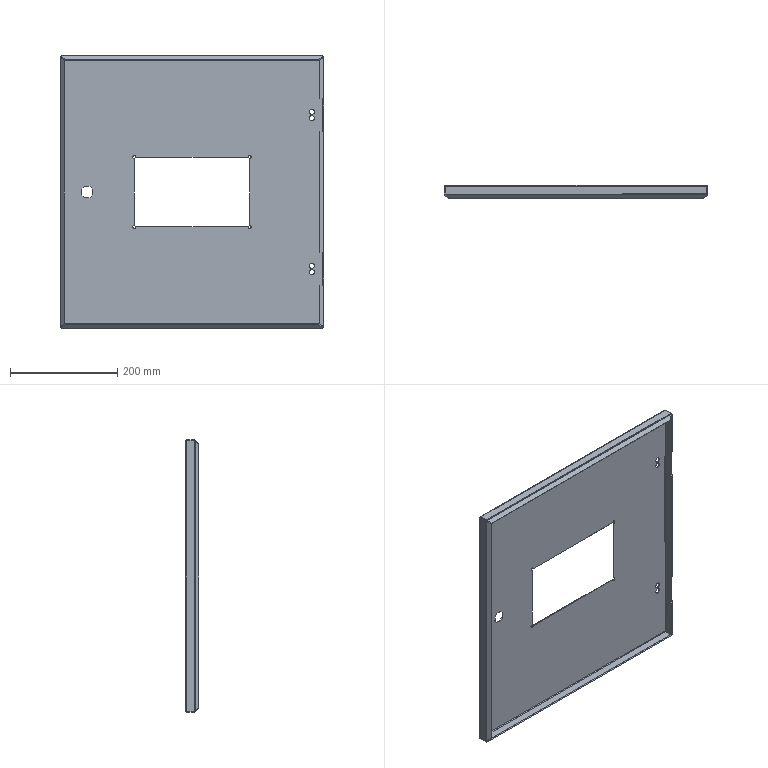Component | SolidWorks | 500CabinetWidthUpperDoor-1 | 1 solid | 114 faces | volume 399839 mm3 | plane 64 | cylinder 34 | spline 16 | commonest cylinder face diameters 5 x10 2 x10 9.5 x8 5.5 x6 | material Plain Carbon Steel